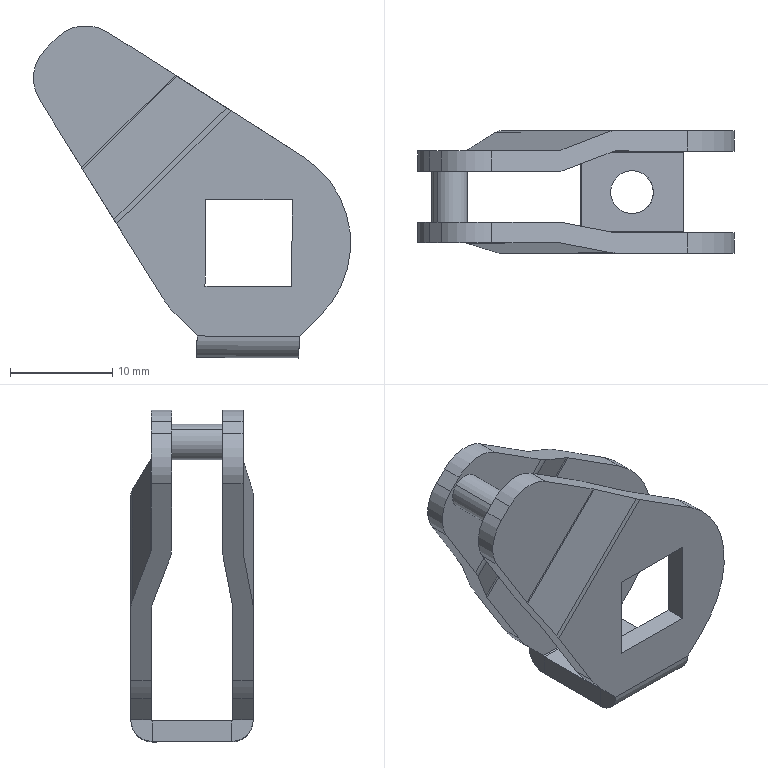Component | SolidWorks | CLS-MechanismOperatingAxisBracketAssembly.SLDPRT-1_CLS-MechanismOperatingAxisBracket-1 | 1 solid | 62 faces | volume 2133 mm3 | plane 38 | cylinder 24 | commonest cylinder face diameters 4.2 x4 2 x4 6 x4 20 x4 8 x4 3.5 x2 0.2 x2